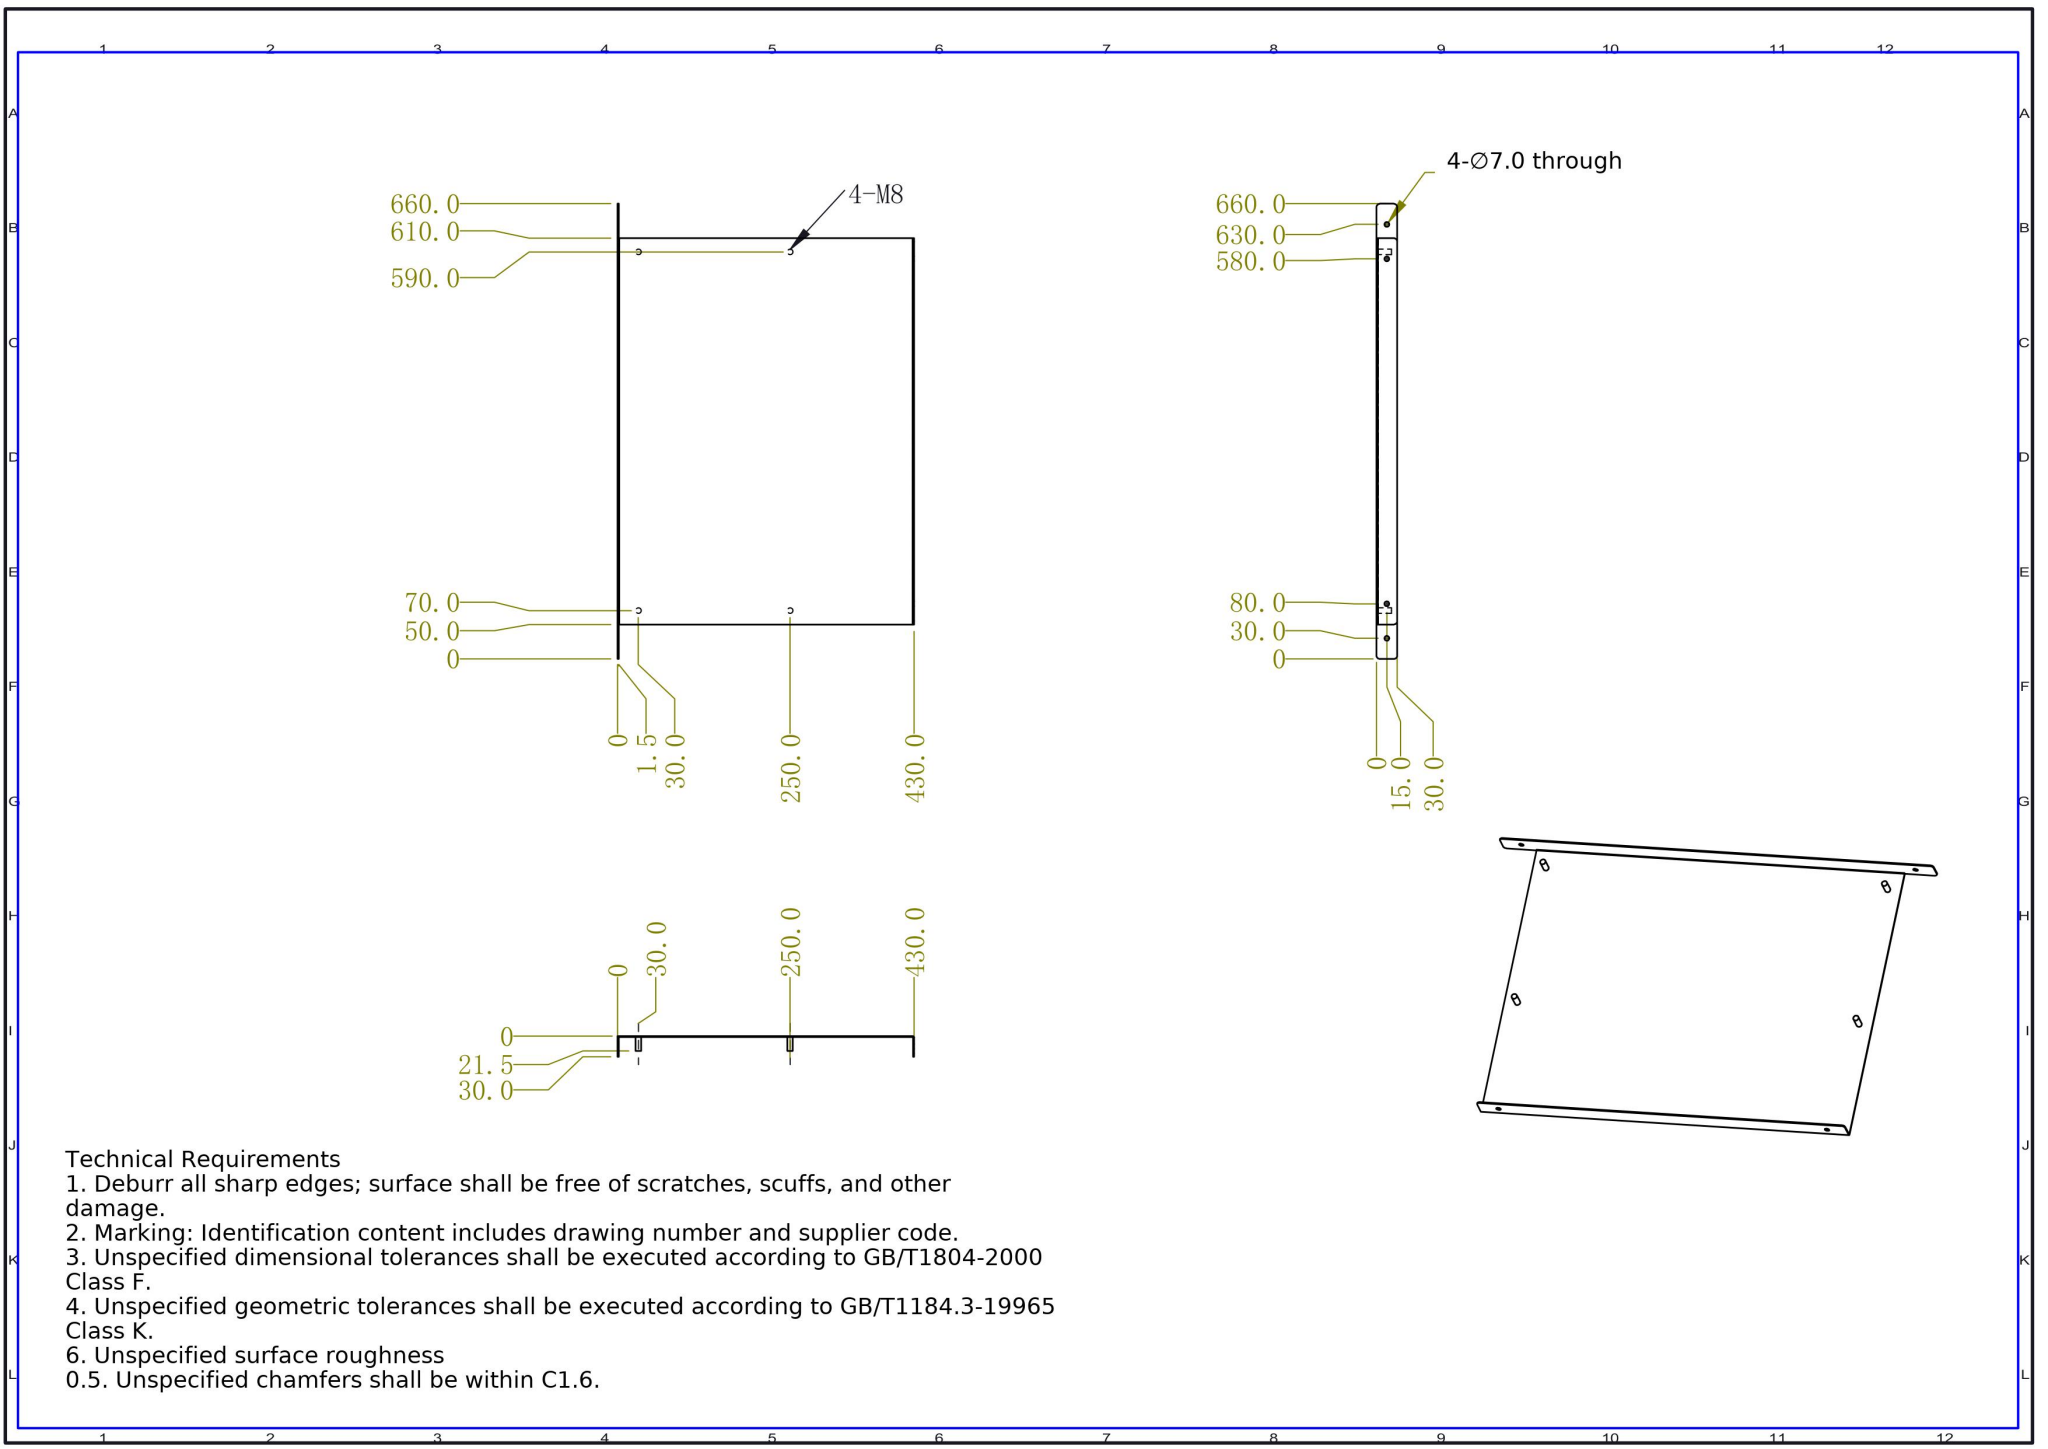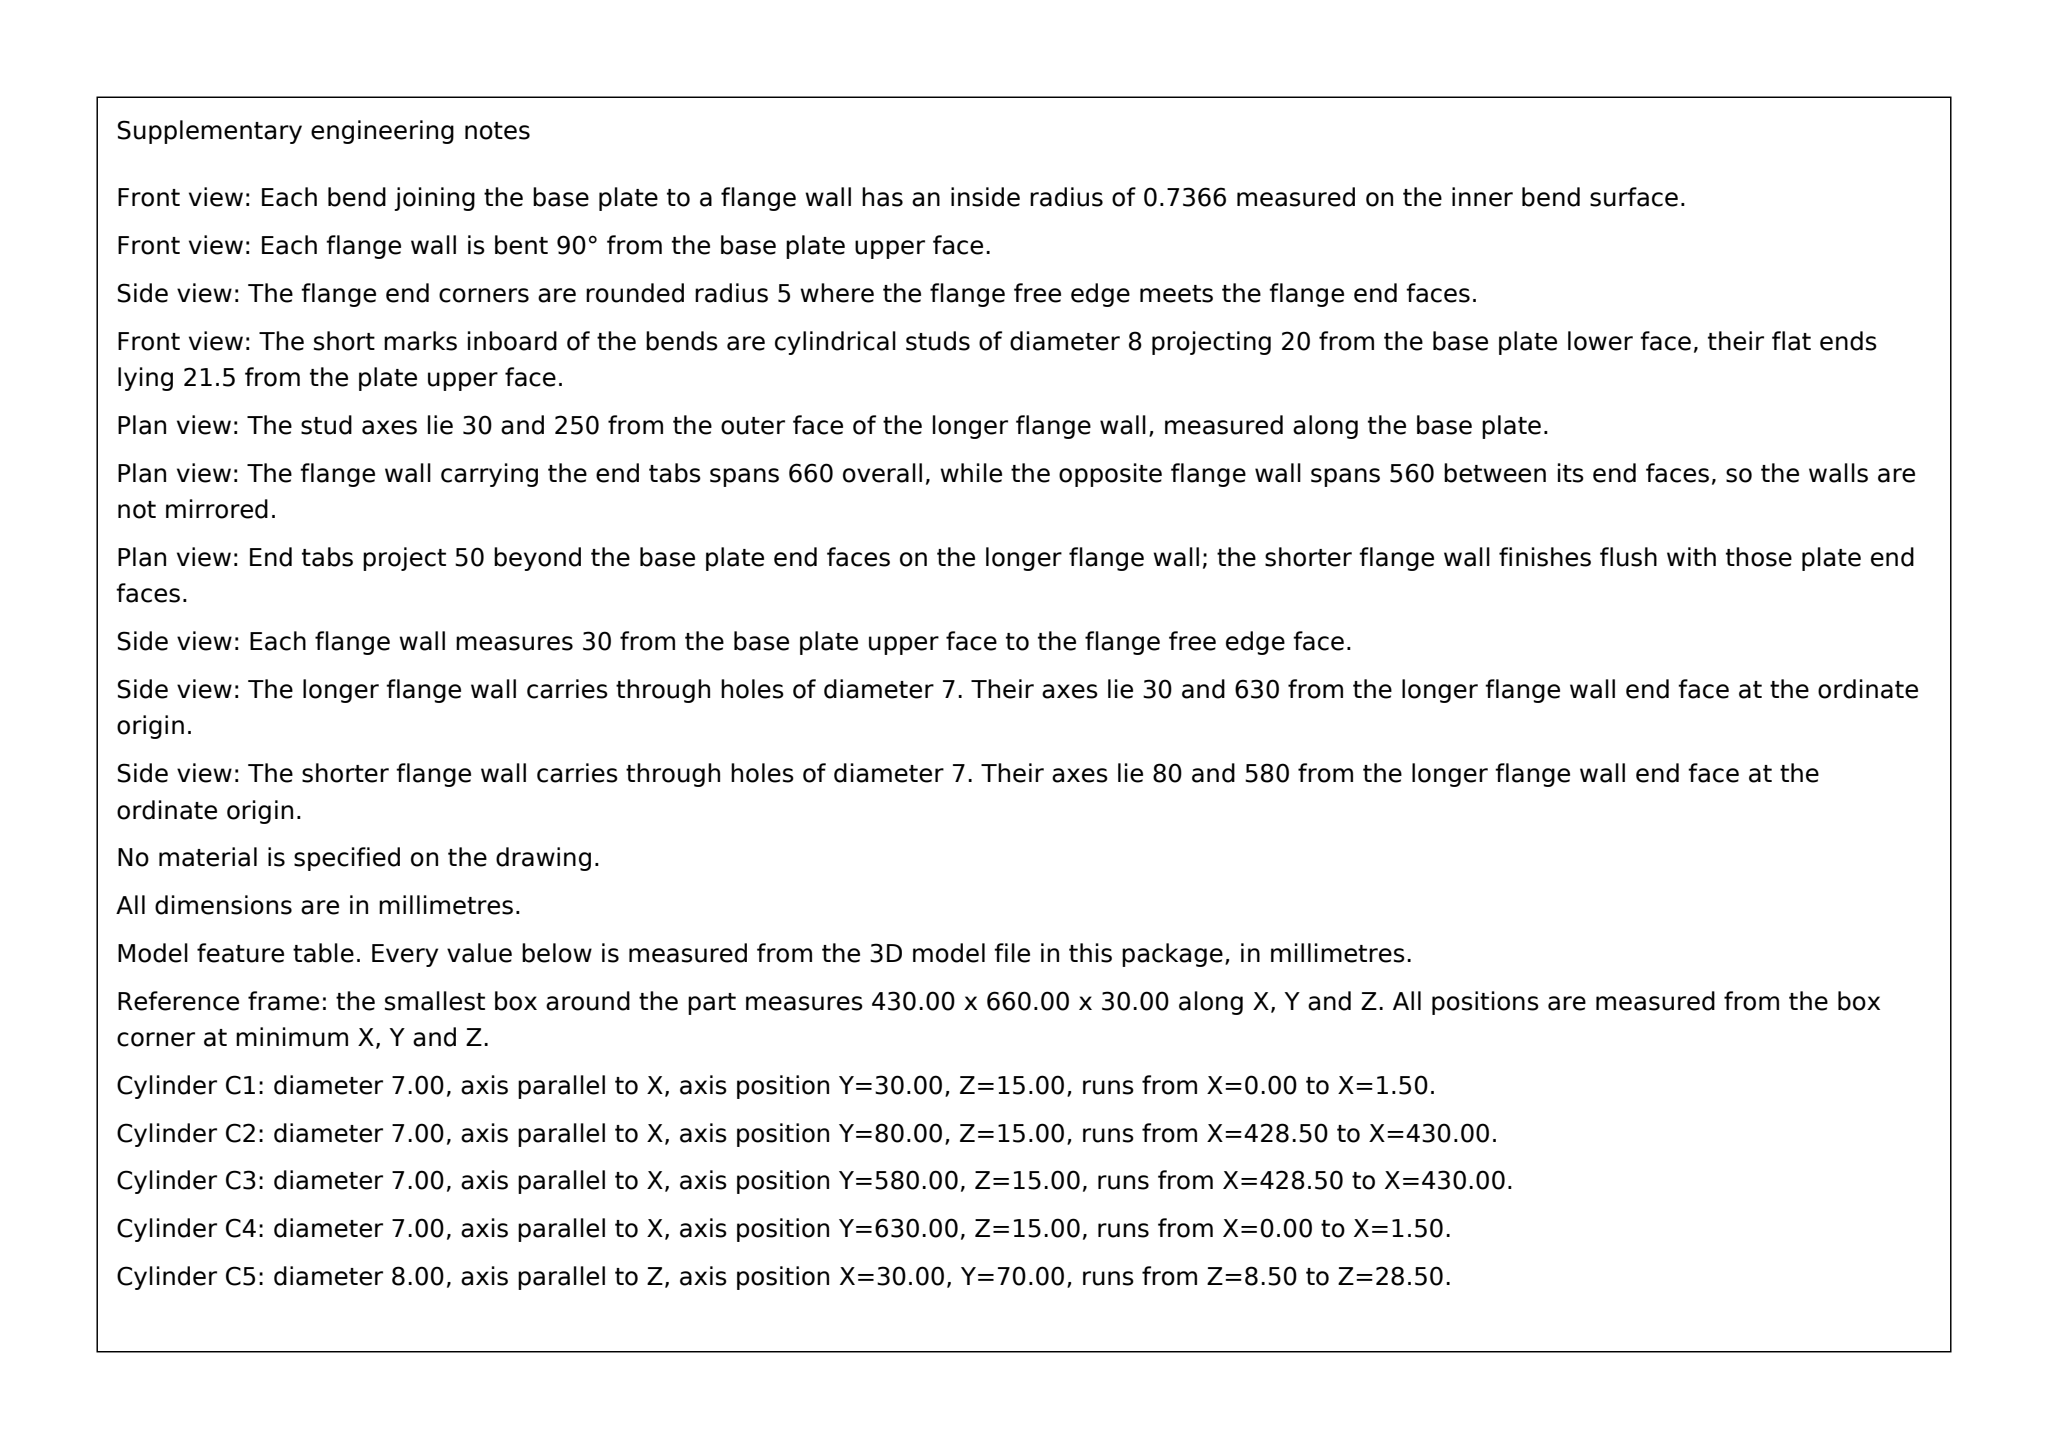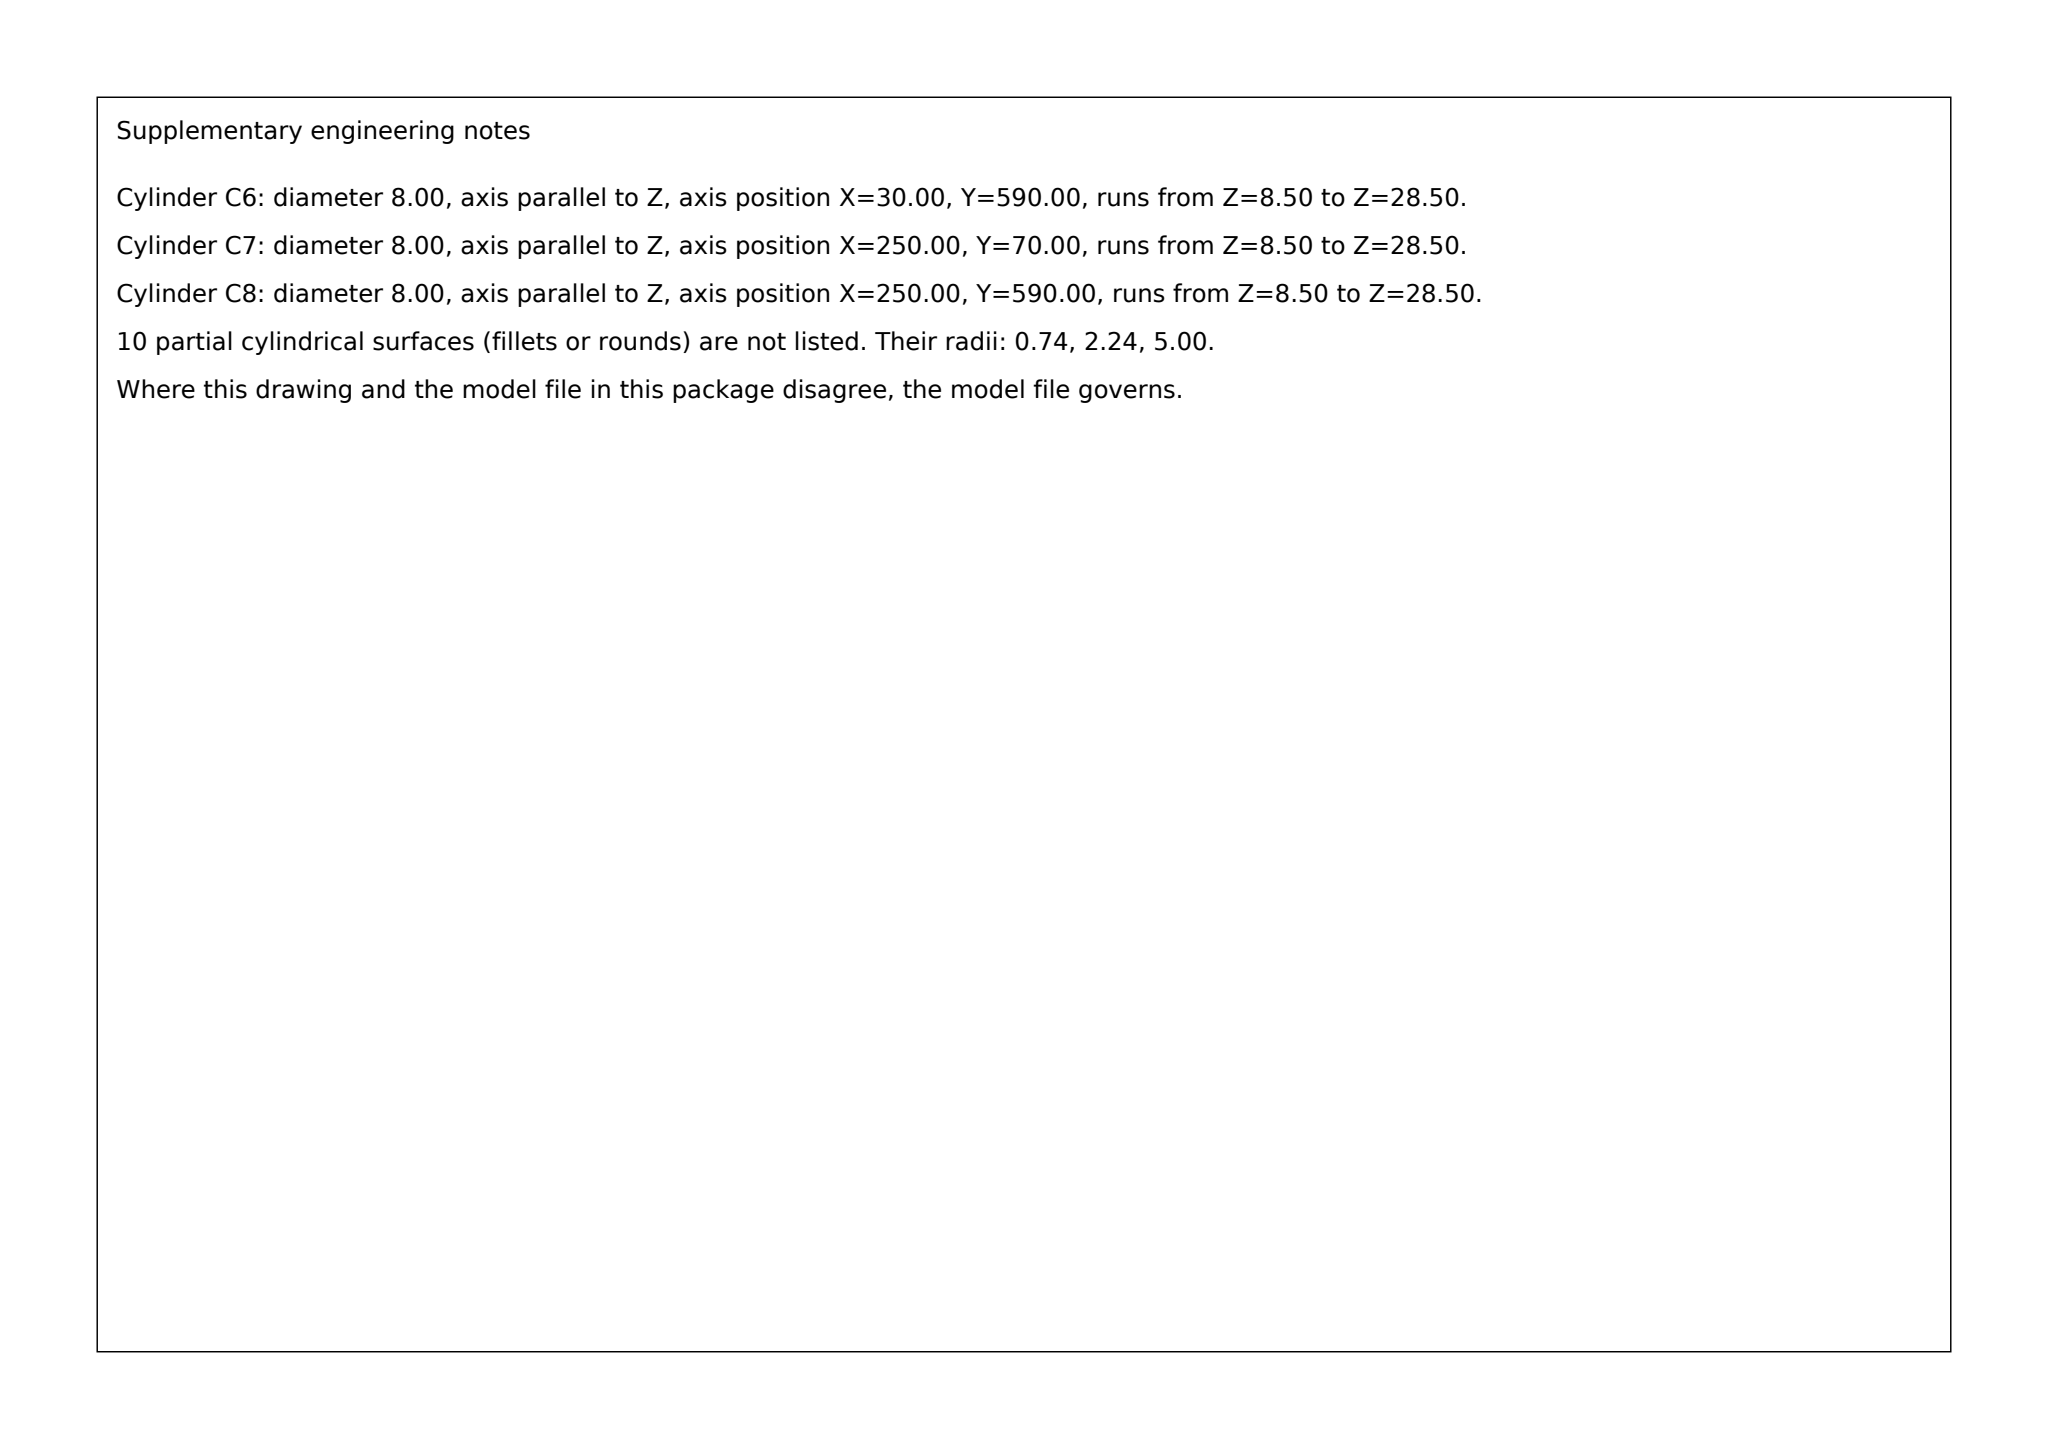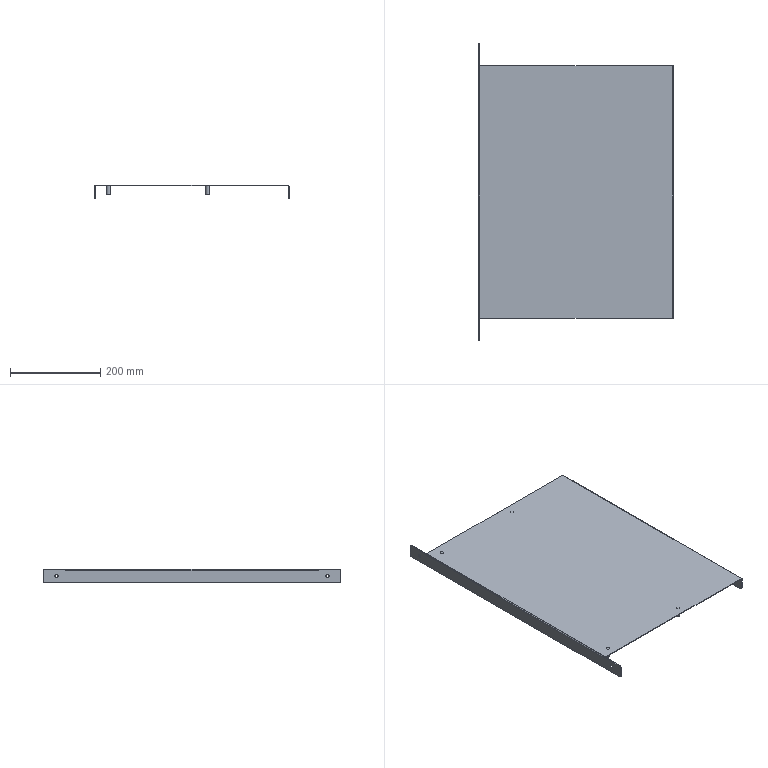Part | SolidWorks | mm | 1 solid | 52 faces | box 430 x 660 x 30 mm | volume 416250 mm3 | cylinder 26 | plane 26 | commonest cylinder face diameters 7 x8 8 x8 10 x6 4.473 x2 1.473 x2